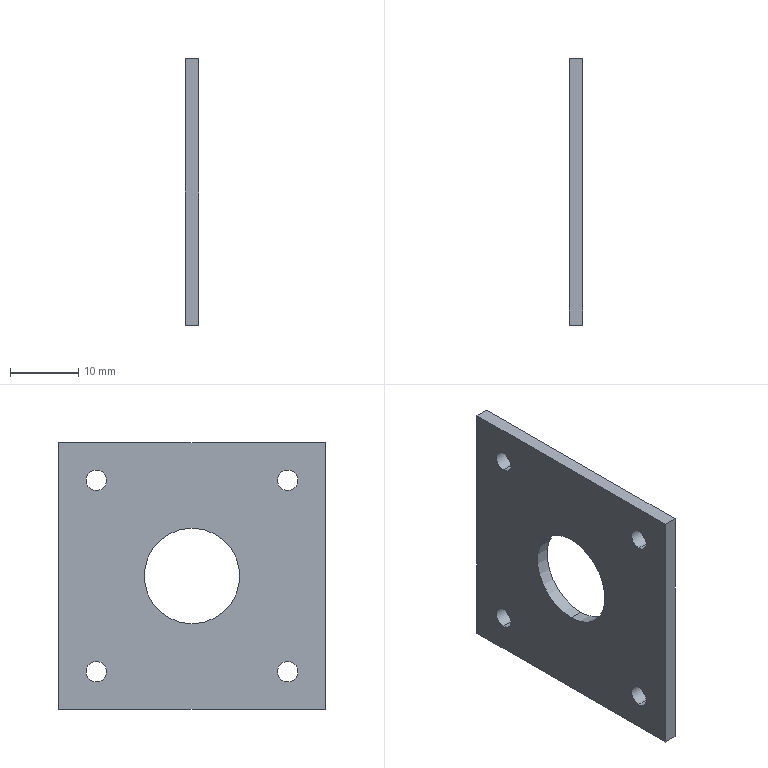Component | SolidWorks | P16BoxWeldment-1_M10WaterproofNutWeldment-10_M10WaterproofStudWeldment-1 | 1 solid | 16 faces | box 2 x 39 x 39 mm | volume 2678 mm3 | cylinder 10 | plane 6 | commonest cylinder face diameters 3 x8 14 x2
STEP:
#1=CARTESIAN_POINT('',(22.309,-7.341,0.6457));
#2=VERTEX_POINT('',#1);
#3=CARTESIAN_POINT('',(22.309,-7.341,0.09449));
#4=VERTEX_POINT('',#3);
#5=CARTESIAN_POINT('',(22.309,-7.341,0.3701));
#6=DIRECTION('',(1.,-0.,0.));
#7=DIRECTION('',(0.,0.,-1.));
#8=AXIS2_PLACEMENT_3D('',#5,#6,#7);
#9=CIRCLE('',#8,0.2756);
#10=EDGE_CURVE('',#2,#4,#9,.T.);
#11=ORIENTED_EDGE('',*,*,#10,.F.);
#12=CARTESIAN_POINT('',(22.388,-7.341,0.6457));
#13=VERTEX_POINT('',#12);
#14=CARTESIAN_POINT('',(22.309,-7.341,0.6457));
#15=DIRECTION('',(1.,-0.,0.));
#16=VECTOR('',#15,39.37);
#17=LINE('',#14,#16);
#18=EDGE_CURVE('',#2,#13,#17,.T.);
#19=ORIENTED_EDGE('',*,*,#18,.T.);
#20=CARTESIAN_POINT('',(22.388,-7.341,0.09449));
#21=VERTEX_POINT('',#20);
#22=CARTESIAN_POINT('',(22.388,-7.341,0.3701));
#23=DIRECTION('',(1.,-0.,0.));
#24=DIRECTION('',(0.,0.,-1.));
#25=AXIS2_PLACEMENT_3D('',#22,#23,#24);
#26=CIRCLE('',#25,0.2756);
#27=EDGE_CURVE('',#13,#21,#26,.T.);
#28=ORIENTED_EDGE('',*,*,#27,.T.);
#29=CARTESIAN_POINT('',(22.309,-7.341,0.09449));
#30=DIRECTION('',(1.,-0.,0.));
#31=VECTOR('',#30,39.37);
#32=LINE('',#29,#31);
#33=EDGE_CURVE('',#4,#21,#32,.T.);
#34=ORIENTED_EDGE('',*,*,#33,.F.);
#35=EDGE_LOOP('',(#11,#19,#28,#34));
#36=FACE_OUTER_BOUND('',#35,.T.);
#37=CARTESIAN_POINT('',(22.309,-7.341,0.3701));
#38=DIRECTION('',(1.,-0.,0.));
#39=DIRECTION('',(0.,0.,-1.));
#40=AXIS2_PLACEMENT_3D('',#37,#38,#39);
#41=CYLINDRICAL_SURFACE('',#40,0.2756);
#42=ADVANCED_FACE('',(#36),#41,.F.);
#43=CARTESIAN_POINT('',(22.309,-7.892,0.9803));
#44=VERTEX_POINT('',#43);
#45=CARTESIAN_POINT('',(22.309,-7.892,0.8622));
#46=VERTEX_POINT('',#45);
#47=CARTESIAN_POINT('',(22.309,-7.892,0.9213));
#48=DIRECTION('',(1.,-0.,0.));
#49=DIRECTION('',(0.,0.,-1.));
#50=AXIS2_PLACEMENT_3D('',#47,#48,#49);
#51=CIRCLE('',#50,0.05906);
#52=EDGE_CURVE('',#44,#46,#51,.T.);
#53=ORIENTED_EDGE('',*,*,#52,.F.);
#54=CARTESIAN_POINT('',(22.388,-7.892,0.9803));
#55=VERTEX_POINT('',#54);
#56=CARTESIAN_POINT('',(22.309,-7.892,0.9803));
#57=DIRECTION('',(1.,-0.,0.));
#58=VECTOR('',#57,39.37);
#59=LINE('',#56,#58);
#60=EDGE_CURVE('',#44,#55,#59,.T.);
#61=ORIENTED_EDGE('',*,*,#60,.T.);
#62=CARTESIAN_POINT('',(22.388,-7.892,0.8622));
#63=VERTEX_POINT('',#62);
#64=CARTESIAN_POINT('',(22.388,-7.892,0.9213));
#65=DIRECTION('',(1.,-0.,0.));
#66=DIRECTION('',(0.,0.,-1.));
#67=AXIS2_PLACEMENT_3D('',#64,#65,#66);
#68=CIRCLE('',#67,0.05906);
#69=EDGE_CURVE('',#55,#63,#68,.T.);
#70=ORIENTED_EDGE('',*,*,#69,.T.);
#71=CARTESIAN_POINT('',(22.309,-7.892,0.8622));
#72=DIRECTION('',(1.,-0.,0.));
#73=VECTOR('',#72,39.37);
#74=LINE('',#71,#73);
#75=EDGE_CURVE('',#46,#63,#74,.T.);
#76=ORIENTED_EDGE('',*,*,#75,.F.);
#77=EDGE_LOOP('',(#53,#61,#70,#76));
#78=FACE_OUTER_BOUND('',#77,.T.);
#79=CARTESIAN_POINT('',(22.309,-7.892,0.9213));
#80=DIRECTION('',(1.,-0.,0.));
#81=DIRECTION('',(0.,0.,-1.));
#82=AXIS2_PLACEMENT_3D('',#79,#80,#81);
#83=CYLINDRICAL_SURFACE('',#82,0.05906);
#84=ADVANCED_FACE('',(#78),#83,.F.);
#85=CARTESIAN_POINT('',(22.309,-7.892,-0.122));
#86=VERTEX_POINT('',#85);
#87=CARTESIAN_POINT('',(22.309,-7.892,-0.2402));
#88=VERTEX_POINT('',#87);
#89=CARTESIAN_POINT('',(22.309,-7.892,-0.1811));
#90=DIRECTION('',(1.,-0.,0.));
#91=DIRECTION('',(0.,0.,-1.));
#92=AXIS2_PLACEMENT_3D('',#89,#90,#91);
#93=CIRCLE('',#92,0.05906);
#94=EDGE_CURVE('',#86,#88,#93,.T.);
#95=ORIENTED_EDGE('',*,*,#94,.F.);
#96=CARTESIAN_POINT('',(22.388,-7.892,-0.122));
#97=VERTEX_POINT('',#96);
#98=CARTESIAN_POINT('',(22.309,-7.892,-0.122));
#99=DIRECTION('',(1.,-0.,0.));
#100=VECTOR('',#99,39.37);
#101=LINE('',#98,#100);
#102=EDGE_CURVE('',#86,#97,#101,.T.);
#103=ORIENTED_EDGE('',*,*,#102,.T.);
#104=CARTESIAN_POINT('',(22.388,-7.892,-0.2402));
#105=VERTEX_POINT('',#104);
#106=CARTESIAN_POINT('',(22.388,-7.892,-0.1811));
#107=DIRECTION('',(1.,-0.,0.));
#108=DIRECTION('',(0.,0.,-1.));
#109=AXIS2_PLACEMENT_3D('',#106,#107,#108);
#110=CIRCLE('',#109,0.05906);
#111=EDGE_CURVE('',#97,#105,#110,.T.);
#112=ORIENTED_EDGE('',*,*,#111,.T.);
#113=CARTESIAN_POINT('',(22.309,-7.892,-0.2402));
#114=DIRECTION('',(1.,-0.,0.));
#115=VECTOR('',#114,39.37);
#116=LINE('',#113,#115);
#117=EDGE_CURVE('',#88,#105,#116,.T.);
#118=ORIENTED_EDGE('',*,*,#117,.F.);
#119=EDGE_LOOP('',(#95,#103,#112,#118));
#120=FACE_OUTER_BOUND('',#119,.T.);
#121=CARTESIAN_POINT('',(22.309,-7.892,-0.1811));
#122=DIRECTION('',(1.,-0.,0.));
#123=DIRECTION('',(0.,0.,-1.));
#124=AXIS2_PLACEMENT_3D('',#121,#122,#123);
#125=CYLINDRICAL_SURFACE('',#124,0.05906);
#126=ADVANCED_FACE('',(#120),#125,.F.);
#127=CARTESIAN_POINT('',(22.309,-6.79,-0.122));
#128=VERTEX_POINT('',#127);
#129=CARTESIAN_POINT('',(22.309,-6.79,-0.2402));
#130=VERTEX_POINT('',#129);
#131=CARTESIAN_POINT('',(22.309,-6.79,-0.1811));
#132=DIRECTION('',(1.,-0.,0.));
#133=DIRECTION('',(0.,0.,-1.));
#134=AXIS2_PLACEMENT_3D('',#131,#132,#133);
#135=CIRCLE('',#134,0.05906);
#136=EDGE_CURVE('',#128,#130,#135,.T.);
#137=ORIENTED_EDGE('',*,*,#136,.F.);
#138=CARTESIAN_POINT('',(22.388,-6.79,-0.122));
#139=VERTEX_POINT('',#138);
#140=CARTESIAN_POINT('',(22.309,-6.79,-0.122));
#141=DIRECTION('',(1.,-0.,0.));
#142=VECTOR('',#141,39.37);
#143=LINE('',#140,#142);
#144=EDGE_CURVE('',#128,#139,#143,.T.);
#145=ORIENTED_EDGE('',*,*,#144,.T.);
#146=CARTESIAN_POINT('',(22.388,-6.79,-0.2402));
#147=VERTEX_POINT('',#146);
#148=CARTESIAN_POINT('',(22.388,-6.79,-0.1811));
#149=DIRECTION('',(1.,-0.,0.));
#150=DIRECTION('',(0.,0.,-1.));
#151=AXIS2_PLACEMENT_3D('',#148,#149,#150);
#152=CIRCLE('',#151,0.05906);
#153=EDGE_CURVE('',#139,#147,#152,.T.);
#154=ORIENTED_EDGE('',*,*,#153,.T.);
#155=CARTESIAN_POINT('',(22.309,-6.79,-0.2402));
#156=DIRECTION('',(1.,-0.,0.));
#157=VECTOR('',#156,39.37);
#158=LINE('',#155,#157);
#159=EDGE_CURVE('',#130,#147,#158,.T.);
#160=ORIENTED_EDGE('',*,*,#159,.F.);
#161=EDGE_LOOP('',(#137,#145,#154,#160));
#162=FACE_OUTER_BOUND('',#161,.T.);
#163=CARTESIAN_POINT('',(22.309,-6.79,-0.1811));
#164=DIRECTION('',(1.,-0.,0.));
#165=DIRECTION('',(0.,0.,-1.));
#166=AXIS2_PLACEMENT_3D('',#163,#164,#165);
#167=CYLINDRICAL_SURFACE('',#166,0.05906);
#168=ADVANCED_FACE('',(#162),#167,.F.);
#169=CARTESIAN_POINT('',(22.309,-6.79,0.9803));
#170=VERTEX_POINT('',#169);
#171=CARTESIAN_POINT('',(22.309,-6.79,0.8622));
#172=VERTEX_POINT('',#171);
#173=CARTESIAN_POINT('',(22.309,-6.79,0.9213));
#174=DIRECTION('',(1.,-0.,0.));
#175=DIRECTION('',(0.,0.,-1.));
#176=AXIS2_PLACEMENT_3D('',#173,#174,#175);
#177=CIRCLE('',#176,0.05906);
#178=EDGE_CURVE('',#170,#172,#177,.T.);
#179=ORIENTED_EDGE('',*,*,#178,.F.);
#180=CARTESIAN_POINT('',(22.388,-6.79,0.9803));
#181=VERTEX_POINT('',#180);
#182=CARTESIAN_POINT('',(22.309,-6.79,0.9803));
#183=DIRECTION('',(1.,-0.,0.));
#184=VECTOR('',#183,39.37);
#185=LINE('',#182,#184);
#186=EDGE_CURVE('',#170,#181,#185,.T.);
#187=ORIENTED_EDGE('',*,*,#186,.T.);
#188=CARTESIAN_POINT('',(22.388,-6.79,0.8622));
#189=VERTEX_POINT('',#188);
#190=CARTESIAN_POINT('',(22.388,-6.79,0.9213));
#191=DIRECTION('',(1.,-0.,0.));
#192=DIRECTION('',(0.,0.,-1.));
#193=AXIS2_PLACEMENT_3D('',#190,#191,#192);
#194=CIRCLE('',#193,0.05906);
#195=EDGE_CURVE('',#181,#189,#194,.T.);
#196=ORIENTED_EDGE('',*,*,#195,.T.);
#197=CARTESIAN_POINT('',(22.309,-6.79,0.8622));
#198=DIRECTION('',(1.,-0.,0.));
#199=VECTOR('',#198,39.37);
#200=LINE('',#197,#199);
#201=EDGE_CURVE('',#172,#189,#200,.T.);
#202=ORIENTED_EDGE('',*,*,#201,.F.);
#203=EDGE_LOOP('',(#179,#187,#196,#202));
#204=FACE_OUTER_BOUND('',#203,.T.);
#205=CARTESIAN_POINT('',(22.309,-6.79,0.9213));
#206=DIRECTION('',(1.,-0.,0.));
#207=DIRECTION('',(0.,0.,-1.));
#208=AXIS2_PLACEMENT_3D('',#205,#206,#207);
#209=CYLINDRICAL_SURFACE('',#208,0.05906);
#210=ADVANCED_FACE('',(#204),#209,.F.);
#211=CARTESIAN_POINT('',(22.388,-8.109,-0.3976));
#212=VERTEX_POINT('',#211);
#213=CARTESIAN_POINT('',(22.388,-6.573,-0.3976));
#214=VERTEX_POINT('',#213);
#215=CARTESIAN_POINT('',(22.388,-8.109,-0.3976));
#216=DIRECTION('',(0.,1.,0.));
#217=VECTOR('',#216,39.37);
#218=LINE('',#215,#217);
#219=EDGE_CURVE('',#212,#214,#218,.T.);
#220=ORIENTED_EDGE('',*,*,#219,.F.);
#221=CARTESIAN_POINT('',(22.309,-8.109,-0.3976));
#222=VERTEX_POINT('',#221);
#223=CARTESIAN_POINT('',(22.309,-8.109,-0.3976));
#224=DIRECTION('',(1.,-0.,0.));
#225=VECTOR('',#224,39.37);
#226=LINE('',#223,#225);
#227=EDGE_CURVE('',#222,#212,#226,.T.);
#228=ORIENTED_EDGE('',*,*,#227,.F.);
#229=CARTESIAN_POINT('',(22.309,-6.573,-0.3976));
#230=VERTEX_POINT('',#229);
#231=CARTESIAN_POINT('',(22.309,-8.109,-0.3976));
#232=DIRECTION('',(0.,1.,0.));
#233=VECTOR('',#232,39.37);
#234=LINE('',#231,#233);
#235=EDGE_CURVE('',#222,#230,#234,.T.);
#236=ORIENTED_EDGE('',*,*,#235,.T.);
#237=CARTESIAN_POINT('',(22.309,-6.573,-0.3976));
#238=DIRECTION('',(1.,-0.,0.));
#239=VECTOR('',#238,39.37);
#240=LINE('',#237,#239);
#241=EDGE_CURVE('',#230,#214,#240,.T.);
#242=ORIENTED_EDGE('',*,*,#241,.T.);
#243=EDGE_LOOP('',(#220,#228,#236,#242));
#244=FACE_OUTER_BOUND('',#243,.T.);
#245=CARTESIAN_POINT('',(22.309,-8.109,-0.3976));
#246=DIRECTION('',(0.,0.,-1.));
#247=DIRECTION('',(-1.,0.,-0.));
#248=AXIS2_PLACEMENT_3D('',#245,#246,#247);
#249=PLANE('',#248);
#250=ADVANCED_FACE('',(#244),#249,.T.);
#251=CARTESIAN_POINT('',(22.388,-8.109,1.138));
#252=VERTEX_POINT('',#251);
#253=CARTESIAN_POINT('',(22.388,-8.109,1.138));
#254=DIRECTION('',(0.,0.,-1.));
#255=VECTOR('',#254,39.37);
#256=LINE('',#253,#255);
#257=EDGE_CURVE('',#252,#212,#256,.T.);
#258=ORIENTED_EDGE('',*,*,#257,.F.);
#259=CARTESIAN_POINT('',(22.309,-8.109,1.138));
#260=VERTEX_POINT('',#259);
#261=CARTESIAN_POINT('',(22.309,-8.109,1.138));
#262=DIRECTION('',(1.,-0.,0.));
#263=VECTOR('',#262,39.37);
#264=LINE('',#261,#263);
#265=EDGE_CURVE('',#260,#252,#264,.T.);
#266=ORIENTED_EDGE('',*,*,#265,.F.);
#267=CARTESIAN_POINT('',(22.309,-8.109,1.138));
#268=DIRECTION('',(0.,0.,-1.));
#269=VECTOR('',#268,39.37);
#270=LINE('',#267,#269);
#271=EDGE_CURVE('',#260,#222,#270,.T.);
#272=ORIENTED_EDGE('',*,*,#271,.T.);
#273=ORIENTED_EDGE('',*,*,#227,.T.);
#274=EDGE_LOOP('',(#258,#266,#272,#273));
#275=FACE_OUTER_BOUND('',#274,.T.);
#276=CARTESIAN_POINT('',(22.309,-8.109,1.138));
#277=DIRECTION('',(-0.,-1.,-0.));
#278=DIRECTION('',(-1.,0.,-0.));
#279=AXIS2_PLACEMENT_3D('',#276,#277,#278);
#280=PLANE('',#279);
#281=ADVANCED_FACE('',(#275),#280,.T.);
#282=CARTESIAN_POINT('',(22.388,-6.573,1.138));
#283=VERTEX_POINT('',#282);
#284=CARTESIAN_POINT('',(22.388,-6.573,1.138));
#285=DIRECTION('',(-0.,-1.,-0.));
#286=VECTOR('',#285,39.37);
#287=LINE('',#284,#286);
#288=EDGE_CURVE('',#283,#252,#287,.T.);
#289=ORIENTED_EDGE('',*,*,#288,.F.);
#290=CARTESIAN_POINT('',(22.309,-6.573,1.138));
#291=VERTEX_POINT('',#290);
#292=CARTESIAN_POINT('',(22.309,-6.573,1.138));
#293=DIRECTION('',(1.,-0.,0.));
#294=VECTOR('',#293,39.37);
#295=LINE('',#292,#294);
#296=EDGE_CURVE('',#291,#283,#295,.T.);
#297=ORIENTED_EDGE('',*,*,#296,.F.);
#298=CARTESIAN_POINT('',(22.309,-6.573,1.138));
#299=DIRECTION('',(-0.,-1.,-0.));
#300=VECTOR('',#299,39.37);
#301=LINE('',#298,#300);
#302=EDGE_CURVE('',#291,#260,#301,.T.);
#303=ORIENTED_EDGE('',*,*,#302,.T.);
#304=ORIENTED_EDGE('',*,*,#265,.T.);
#305=EDGE_LOOP('',(#289,#297,#303,#304));
#306=FACE_OUTER_BOUND('',#305,.T.);
#307=CARTESIAN_POINT('',(22.309,-6.573,1.138));
#308=DIRECTION('',(-0.,0.,1.));
#309=DIRECTION('',(1.,-0.,0.));
#310=AXIS2_PLACEMENT_3D('',#307,#308,#309);
#311=PLANE('',#310);
#312=ADVANCED_FACE('',(#306),#311,.T.);
#313=CARTESIAN_POINT('',(22.388,-6.573,-0.3976));
#314=DIRECTION('',(-0.,0.,1.));
#315=VECTOR('',#314,39.37);
#316=LINE('',#313,#315);
#317=EDGE_CURVE('',#214,#283,#316,.T.);
#318=ORIENTED_EDGE('',*,*,#317,.F.);
#319=ORIENTED_EDGE('',*,*,#241,.F.);
#320=CARTESIAN_POINT('',(22.309,-6.573,-0.3976));
#321=DIRECTION('',(-0.,0.,1.));
#322=VECTOR('',#321,39.37);
#323=LINE('',#320,#322);
#324=EDGE_CURVE('',#230,#291,#323,.T.);
#325=ORIENTED_EDGE('',*,*,#324,.T.);
#326=ORIENTED_EDGE('',*,*,#296,.T.);
#327=EDGE_LOOP('',(#318,#319,#325,#326));
#328=FACE_OUTER_BOUND('',#327,.T.);
#329=CARTESIAN_POINT('',(22.309,-6.573,-0.3976));
#330=DIRECTION('',(0.,1.,0.));
#331=DIRECTION('',(1.,-0.,0.));
#332=AXIS2_PLACEMENT_3D('',#329,#330,#331);
#333=PLANE('',#332);
#334=ADVANCED_FACE('',(#328),#333,.T.);
#335=CARTESIAN_POINT('',(22.309,-7.341,0.3701));
#336=DIRECTION('',(1.,-0.,0.));
#337=DIRECTION('',(0.,0.,-1.));
#338=AXIS2_PLACEMENT_3D('',#335,#336,#337);
#339=CIRCLE('',#338,0.2756);
#340=EDGE_CURVE('',#4,#2,#339,.T.);
#341=ORIENTED_EDGE('',*,*,#340,.T.);
#342=ORIENTED_EDGE('',*,*,#10,.T.);
#343=EDGE_LOOP('',(#341,#342));
#344=FACE_BOUND('',#343,.T.);
#345=CARTESIAN_POINT('',(22.309,-7.892,0.9213));
#346=DIRECTION('',(1.,-0.,0.));
#347=DIRECTION('',(0.,0.,-1.));
#348=AXIS2_PLACEMENT_3D('',#345,#346,#347);
#349=CIRCLE('',#348,0.05906);
#350=EDGE_CURVE('',#46,#44,#349,.T.);
#351=ORIENTED_EDGE('',*,*,#350,.T.);
#352=ORIENTED_EDGE('',*,*,#52,.T.);
#353=EDGE_LOOP('',(#351,#352));
#354=FACE_BOUND('',#353,.T.);
#355=CARTESIAN_POINT('',(22.309,-7.892,-0.1811));
#356=DIRECTION('',(1.,-0.,0.));
#357=DIRECTION('',(0.,0.,-1.));
#358=AXIS2_PLACEMENT_3D('',#355,#356,#357);
#359=CIRCLE('',#358,0.05906);
#360=EDGE_CURVE('',#88,#86,#359,.T.);
#361=ORIENTED_EDGE('',*,*,#360,.T.);
#362=ORIENTED_EDGE('',*,*,#94,.T.);
#363=EDGE_LOOP('',(#361,#362));
#364=FACE_BOUND('',#363,.T.);
#365=CARTESIAN_POINT('',(22.309,-6.79,-0.1811));
#366=DIRECTION('',(1.,-0.,0.));
#367=DIRECTION('',(0.,0.,-1.));
#368=AXIS2_PLACEMENT_3D('',#365,#366,#367);
#369=CIRCLE('',#368,0.05906);
#370=EDGE_CURVE('',#130,#128,#369,.T.);
#371=ORIENTED_EDGE('',*,*,#370,.T.);
#372=ORIENTED_EDGE('',*,*,#136,.T.);
#373=EDGE_LOOP('',(#371,#372));
#374=FACE_BOUND('',#373,.T.);
#375=CARTESIAN_POINT('',(22.309,-6.79,0.9213));
#376=DIRECTION('',(1.,-0.,0.));
#377=DIRECTION('',(0.,0.,-1.));
#378=AXIS2_PLACEMENT_3D('',#375,#376,#377);
#379=CIRCLE('',#378,0.05906);
#380=EDGE_CURVE('',#172,#170,#379,.T.);
#381=ORIENTED_EDGE('',*,*,#380,.T.);
#382=ORIENTED_EDGE('',*,*,#178,.T.);
#383=EDGE_LOOP('',(#381,#382));
#384=FACE_BOUND('',#383,.T.);
#385=ORIENTED_EDGE('',*,*,#235,.F.);
#386=ORIENTED_EDGE('',*,*,#271,.F.);
#387=ORIENTED_EDGE('',*,*,#302,.F.);
#388=ORIENTED_EDGE('',*,*,#324,.F.);
#389=EDGE_LOOP('',(#385,#386,#387,#388));
#390=FACE_OUTER_BOUND('',#389,.T.);
#391=CARTESIAN_POINT('',(22.309,-7.341,0.3701));
#392=DIRECTION('',(1.,-0.,0.));
#393=DIRECTION('',(0.,0.,-1.));
#394=AXIS2_PLACEMENT_3D('',#391,#392,#393);
#395=PLANE('',#394);
#396=ADVANCED_FACE('',(#344,#354,#364,#374,#384,#390),#395,.F.);
#397=CARTESIAN_POINT('',(22.388,-7.341,0.3701));
#398=DIRECTION('',(1.,-0.,0.));
#399=DIRECTION('',(0.,0.,-1.));
#400=AXIS2_PLACEMENT_3D('',#397,#398,#399);
#401=CIRCLE('',#400,0.2756);
#402=EDGE_CURVE('',#21,#13,#401,.T.);
#403=ORIENTED_EDGE('',*,*,#402,.F.);
#404=ORIENTED_EDGE('',*,*,#27,.F.);
#405=EDGE_LOOP('',(#403,#404));
#406=FACE_BOUND('',#405,.T.);
#407=CARTESIAN_POINT('',(22.388,-7.892,0.9213));
#408=DIRECTION('',(1.,-0.,0.));
#409=DIRECTION('',(0.,0.,-1.));
#410=AXIS2_PLACEMENT_3D('',#407,#408,#409);
#411=CIRCLE('',#410,0.05906);
#412=EDGE_CURVE('',#63,#55,#411,.T.);
#413=ORIENTED_EDGE('',*,*,#412,.F.);
#414=ORIENTED_EDGE('',*,*,#69,.F.);
#415=EDGE_LOOP('',(#413,#414));
#416=FACE_BOUND('',#415,.T.);
#417=CARTESIAN_POINT('',(22.388,-7.892,-0.1811));
#418=DIRECTION('',(1.,-0.,0.));
#419=DIRECTION('',(0.,0.,-1.));
#420=AXIS2_PLACEMENT_3D('',#417,#418,#419);
#421=CIRCLE('',#420,0.05906);
#422=EDGE_CURVE('',#105,#97,#421,.T.);
#423=ORIENTED_EDGE('',*,*,#422,.F.);
#424=ORIENTED_EDGE('',*,*,#111,.F.);
#425=EDGE_LOOP('',(#423,#424));
#426=FACE_BOUND('',#425,.T.);
#427=CARTESIAN_POINT('',(22.388,-6.79,-0.1811));
#428=DIRECTION('',(1.,-0.,0.));
#429=DIRECTION('',(0.,0.,-1.));
#430=AXIS2_PLACEMENT_3D('',#427,#428,#429);
#431=CIRCLE('',#430,0.05906);
#432=EDGE_CURVE('',#147,#139,#431,.T.);
#433=ORIENTED_EDGE('',*,*,#432,.F.);
#434=ORIENTED_EDGE('',*,*,#153,.F.);
#435=EDGE_LOOP('',(#433,#434));
#436=FACE_BOUND('',#435,.T.);
#437=CARTESIAN_POINT('',(22.388,-6.79,0.9213));
#438=DIRECTION('',(1.,-0.,0.));
#439=DIRECTION('',(0.,0.,-1.));
#440=AXIS2_PLACEMENT_3D('',#437,#438,#439);
#441=CIRCLE('',#440,0.05906);
#442=EDGE_CURVE('',#189,#181,#441,.T.);
#443=ORIENTED_EDGE('',*,*,#442,.F.);
#444=ORIENTED_EDGE('',*,*,#195,.F.);
#445=EDGE_LOOP('',(#443,#444));
#446=FACE_BOUND('',#445,.T.);
#447=ORIENTED_EDGE('',*,*,#219,.T.);
#448=ORIENTED_EDGE('',*,*,#317,.T.);
#449=ORIENTED_EDGE('',*,*,#288,.T.);
#450=ORIENTED_EDGE('',*,*,#257,.T.);
#451=EDGE_LOOP('',(#447,#448,#449,#450));
#452=FACE_OUTER_BOUND('',#451,.T.);
#453=CARTESIAN_POINT('',(22.388,-7.341,0.3701));
#454=DIRECTION('',(1.,-0.,0.));
#455=DIRECTION('',(0.,0.,-1.));
#456=AXIS2_PLACEMENT_3D('',#453,#454,#455);
#457=PLANE('',#456);
#458=ADVANCED_FACE('',(#406,#416,#426,#436,#446,#452),#457,.T.);
#459=ORIENTED_EDGE('',*,*,#186,.F.);
#460=ORIENTED_EDGE('',*,*,#380,.F.);
#461=ORIENTED_EDGE('',*,*,#201,.T.);
#462=ORIENTED_EDGE('',*,*,#442,.T.);
#463=EDGE_LOOP('',(#459,#460,#461,#462));
#464=FACE_OUTER_BOUND('',#463,.T.);
#465=CARTESIAN_POINT('',(22.309,-6.79,0.9213));
#466=DIRECTION('',(1.,-0.,0.));
#467=DIRECTION('',(0.,0.,-1.));
#468=AXIS2_PLACEMENT_3D('',#465,#466,#467);
#469=CYLINDRICAL_SURFACE('',#468,0.05906);
#470=ADVANCED_FACE('',(#464),#469,.F.);
#471=ORIENTED_EDGE('',*,*,#144,.F.);
#472=ORIENTED_EDGE('',*,*,#370,.F.);
#473=ORIENTED_EDGE('',*,*,#159,.T.);
#474=ORIENTED_EDGE('',*,*,#432,.T.);
#475=EDGE_LOOP('',(#471,#472,#473,#474));
#476=FACE_OUTER_BOUND('',#475,.T.);
#477=CARTESIAN_POINT('',(22.309,-6.79,-0.1811));
#478=DIRECTION('',(1.,-0.,0.));
#479=DIRECTION('',(0.,0.,-1.));
#480=AXIS2_PLACEMENT_3D('',#477,#478,#479);
#481=CYLINDRICAL_SURFACE('',#480,0.05906);
#482=ADVANCED_FACE('',(#476),#481,.F.);
#483=ORIENTED_EDGE('',*,*,#102,.F.);
#484=ORIENTED_EDGE('',*,*,#360,.F.);
#485=ORIENTED_EDGE('',*,*,#117,.T.);
#486=ORIENTED_EDGE('',*,*,#422,.T.);
#487=EDGE_LOOP('',(#483,#484,#485,#486));
#488=FACE_OUTER_BOUND('',#487,.T.);
#489=CARTESIAN_POINT('',(22.309,-7.892,-0.1811));
#490=DIRECTION('',(1.,-0.,0.));
#491=DIRECTION('',(0.,0.,-1.));
#492=AXIS2_PLACEMENT_3D('',#489,#490,#491);
#493=CYLINDRICAL_SURFACE('',#492,0.05906);
#494=ADVANCED_FACE('',(#488),#493,.F.);
#495=ORIENTED_EDGE('',*,*,#60,.F.);
#496=ORIENTED_EDGE('',*,*,#350,.F.);
#497=ORIENTED_EDGE('',*,*,#75,.T.);
#498=ORIENTED_EDGE('',*,*,#412,.T.);
#499=EDGE_LOOP('',(#495,#496,#497,#498));
#500=FACE_OUTER_BOUND('',#499,.T.);
#501=CARTESIAN_POINT('',(22.309,-7.892,0.9213));
#502=DIRECTION('',(1.,-0.,0.));
#503=DIRECTION('',(0.,0.,-1.));
#504=AXIS2_PLACEMENT_3D('',#501,#502,#503);
#505=CYLINDRICAL_SURFACE('',#504,0.05906);
#506=ADVANCED_FACE('',(#500),#505,.F.);
#507=ORIENTED_EDGE('',*,*,#18,.F.);
#508=ORIENTED_EDGE('',*,*,#340,.F.);
#509=ORIENTED_EDGE('',*,*,#33,.T.);
#510=ORIENTED_EDGE('',*,*,#402,.T.);
#511=EDGE_LOOP('',(#507,#508,#509,#510));
#512=FACE_OUTER_BOUND('',#511,.T.);
#513=CARTESIAN_POINT('',(22.309,-7.341,0.3701));
#514=DIRECTION('',(1.,-0.,0.));
#515=DIRECTION('',(0.,0.,-1.));
#516=AXIS2_PLACEMENT_3D('',#513,#514,#515);
#517=CYLINDRICAL_SURFACE('',#516,0.2756);
#518=ADVANCED_FACE('',(#512),#517,.F.);
#519=CLOSED_SHELL('',(#42,#84,#126,#168,#210,#250,#281,#312,#334,#396,#458,#470,#482,#494,#506,#518));
#520=MANIFOLD_SOLID_BREP('',#519);
#521=CARTESIAN_POINT('',(0.,0.,0.));
#522=DIRECTION('',(0.,0.,1.));
#523=DIRECTION('',(1.,0.,0.));
#524=AXIS2_PLACEMENT_3D('',#521,#522,#523);
#525=(LENGTH_UNIT()NAMED_UNIT(*)SI_UNIT($,.METRE.));
#526=LENGTH_MEASURE_WITH_UNIT(LENGTH_MEASURE(0.0254),#525);
#527=DIMENSIONAL_EXPONENTS(1.,0.,0.,0.,0.,0.,0.);
#528=(CONVERSION_BASED_UNIT('',#526)LENGTH_UNIT()NAMED_UNIT(#527));
#529=UNCERTAINTY_MEASURE_WITH_UNIT(LENGTH_MEASURE(0.00001),#528,'','');
#530=(NAMED_UNIT(*)PLANE_ANGLE_UNIT()SI_UNIT($,.RADIAN.));
#531=(NAMED_UNIT(*)SI_UNIT($,.STERADIAN.)SOLID_ANGLE_UNIT());
#532=(GEOMETRIC_REPRESENTATION_CONTEXT(3)GLOBAL_UNCERTAINTY_ASSIGNED_CONTEXT((#529))GLOBAL_UNIT_ASSIGNED_CONTEXT((#528,#530,#531))REPRESENTATION_CONTEXT('',''));
#533=ADVANCED_BREP_SHAPE_REPRESENTATION('',(#520,#524),#532);
#534=COLOUR_RGB('',0.7922,0.8196,0.9333);
#535=FILL_AREA_STYLE_COLOUR('',#534);
#536=FILL_AREA_STYLE('',(#535));
#537=SURFACE_STYLE_FILL_AREA(#536);
#538=SURFACE_SIDE_STYLE('',(#537));
#539=SURFACE_STYLE_USAGE(.BOTH.,#538);
#540=PRESENTATION_STYLE_ASSIGNMENT((#539));
#541=STYLED_ITEM('',(#540),#520);
#542=PRESENTATION_LAYER_ASSIGNMENT('','',(#541));
#543=(LENGTH_UNIT()NAMED_UNIT(*)SI_UNIT($,.METRE.));
#544=LENGTH_MEASURE_WITH_UNIT(LENGTH_MEASURE(0.0254),#543);
#545=DIMENSIONAL_EXPONENTS(1.,0.,0.,0.,0.,0.,0.);
#546=(CONVERSION_BASED_UNIT('',#544)LENGTH_UNIT()NAMED_UNIT(#545));
#547=UNCERTAINTY_MEASURE_WITH_UNIT(LENGTH_MEASURE(0.00001),#546,'','');
#548=(NAMED_UNIT(*)PLANE_ANGLE_UNIT()SI_UNIT($,.RADIAN.));
#549=(NAMED_UNIT(*)SI_UNIT($,.STERADIAN.)SOLID_ANGLE_UNIT());
#550=(GEOMETRIC_REPRESENTATION_CONTEXT(3)GLOBAL_UNCERTAINTY_ASSIGNED_CONTEXT((#547))GLOBAL_UNIT_ASSIGNED_CONTEXT((#546,#548,#549))REPRESENTATION_CONTEXT('',''));
#551=MECHANICAL_DESIGN_GEOMETRIC_PRESENTATION_REPRESENTATION('',(#541),#550);